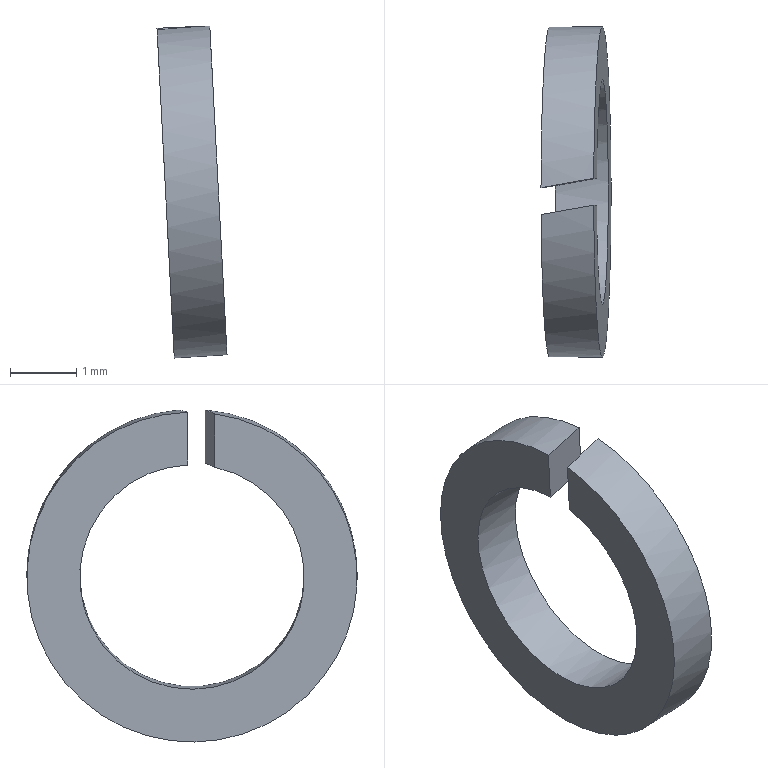Component | NX | GB93-87_3 | 1 solid | 6 faces | box 1.06 x 5 x 5.03 mm | volume 8 mm3 | plane 4 | cylinder 2 | commonest cylinder face diameters 5 x1 3.4 x1
STEP:
#1=CARTESIAN_POINT('',(0.,0.,0.));
#2=DIRECTION('',(0.,0.,1.));
#3=DIRECTION('',(1.,0.,0.));
#4=AXIS2_PLACEMENT_3D('',#1,#2,#3);
#5=CARTESIAN_POINT('',(4.816,-45.247,162.495));
#6=VERTEX_POINT('',#5);
#7=CARTESIAN_POINT('',(4.816,-44.841,162.495));
#8=VERTEX_POINT('',#7);
#9=CARTESIAN_POINT('',(4.947,-45.044,160.007));
#10=DIRECTION('',(0.9986,0.,0.05234));
#11=DIRECTION('',(0.05234,0.,-0.9986));
#12=AXIS2_PLACEMENT_3D('',#9,#10,#11);
#13=CIRCLE('',#12,2.5);
#14=CARTESIAN_POINT('',(4.947,-45.044,160.007));
#15=DIRECTION('',(0.9986,0.,0.05234));
#16=DIRECTION('',(0.05234,0.,-0.9986));
#17=AXIS2_PLACEMENT_3D('',#14,#15,#16);
#18=CYLINDRICAL_SURFACE('',#17,2.5);
#19=CARTESIAN_POINT('',(-6.283,0.));
#20=DIRECTION('',(1.,0.));
#21=VECTOR('',#20,1.);
#22=LINE('',#19,#21);
#23=(GEOMETRIC_REPRESENTATION_CONTEXT(2)PARAMETRIC_REPRESENTATION_CONTEXT()REPRESENTATION_CONTEXT('',''));
#24=DEFINITIONAL_REPRESENTATION('',(#22),#23);
#25=PCURVE('',#18,#24);
#26=CARTESIAN_POINT('',(4.947,-43.344,160.007));
#27=DIRECTION('',(0.9986,0.,0.05234));
#28=DIRECTION('',(0.05234,0.,-0.9986));
#29=AXIS2_PLACEMENT_3D('',#26,#27,#28);
#30=PLANE('',#29);
#31=CARTESIAN_POINT('',(0.,-1.7));
#32=DIRECTION('',(1.,0.));
#33=AXIS2_PLACEMENT_2D('',#31,#32);
#34=CIRCLE('',#33,2.5);
#35=(GEOMETRIC_REPRESENTATION_CONTEXT(2)PARAMETRIC_REPRESENTATION_CONTEXT()REPRESENTATION_CONTEXT('',''));
#36=DEFINITIONAL_REPRESENTATION('',(#34),#35);
#37=PCURVE('',#30,#36);
#38=SURFACE_CURVE('',#13,(#25,#37),.PCURVE_S1.);
#39=EDGE_CURVE('',#6,#8,#38,.T.);
#40=ORIENTED_EDGE('',*,*,#39,.F.);
#41=CARTESIAN_POINT('',(4.018,-45.388,162.438));
#42=VERTEX_POINT('',#41);
#43=CARTESIAN_POINT('',(6.097,-45.044,160.067));
#44=DIRECTION('',(0.1734,-0.9848,0.009088));
#45=DIRECTION('',(0.9835,0.1736,0.05154));
#46=AXIS2_PLACEMENT_3D('',#43,#44,#45);
#47=ELLIPSE('',#46,14.397,2.5);
#48=CARTESIAN_POINT('',(-3.06,-0.));
#49=CARTESIAN_POINT('',(-3.003,-0.8));
#50=B_SPLINE_CURVE_WITH_KNOTS('',1,(#48,#49),.UNSPECIFIED.,.F.,.F.,(2,2),(1.652,1.709),.PIECEWISE_BEZIER_KNOTS.);
#51=(GEOMETRIC_REPRESENTATION_CONTEXT(2)PARAMETRIC_REPRESENTATION_CONTEXT()REPRESENTATION_CONTEXT('',''));
#52=DEFINITIONAL_REPRESENTATION('',(#50),#51);
#53=PCURVE('',#18,#52);
#54=CARTESIAN_POINT('',(3.605,-45.449,163.692));
#55=DIRECTION('',(-0.1734,0.9848,-0.009088));
#56=DIRECTION('',(-0.9835,-0.1736,-0.05154));
#57=AXIS2_PLACEMENT_3D('',#54,#55,#56);
#58=PLANE('',#57);
#59=CARTESIAN_POINT('',(-16.731,-3.75));
#60=CARTESIAN_POINT('',(-16.731,0.5801));
#61=CARTESIAN_POINT('',(4.864,-1.585));
#62=CARTESIAN_POINT('',(26.46,-3.75));
#63=CARTESIAN_POINT('',(4.864,-5.915));
#64=CARTESIAN_POINT('',(-16.731,-8.08));
#65=CARTESIAN_POINT('',(-16.731,-3.75));
#66=(BOUNDED_CURVE()B_SPLINE_CURVE(2,(#59,#60,#61,#62,#63,#64,#65),.UNSPECIFIED.,.T.,.F.)B_SPLINE_CURVE_WITH_KNOTS((1,2,2,2,2,1),(-2.094,0.,2.094,4.189,6.283,8.378),.UNSPECIFIED.)CURVE()GEOMETRIC_REPRESENTATION_ITEM()RATIONAL_B_SPLINE_CURVE((1.,0.5,1.,0.5,1.,0.5,1.))REPRESENTATION_ITEM(''));
#67=(GEOMETRIC_REPRESENTATION_CONTEXT(2)PARAMETRIC_REPRESENTATION_CONTEXT()REPRESENTATION_CONTEXT('',''));
#68=DEFINITIONAL_REPRESENTATION('',(#66),#67);
#69=PCURVE('',#58,#68);
#70=SURFACE_CURVE('',#47,(#53,#69),.PCURVE_S1.);
#71=EDGE_CURVE('',#6,#42,#70,.T.);
#72=ORIENTED_EDGE('',*,*,#71,.T.);
#73=CARTESIAN_POINT('',(4.017,-44.982,162.461));
#74=VERTEX_POINT('',#73);
#75=CARTESIAN_POINT('',(4.148,-45.044,159.965));
#76=DIRECTION('',(0.9986,0.,0.05234));
#77=DIRECTION('',(0.05234,0.,-0.9986));
#78=AXIS2_PLACEMENT_3D('',#75,#76,#77);
#79=CIRCLE('',#78,2.5);
#80=CARTESIAN_POINT('',(-6.283,-0.8));
#81=DIRECTION('',(1.,-0.));
#82=VECTOR('',#81,1.);
#83=LINE('',#80,#82);
#84=(GEOMETRIC_REPRESENTATION_CONTEXT(2)PARAMETRIC_REPRESENTATION_CONTEXT()REPRESENTATION_CONTEXT('',''));
#85=DEFINITIONAL_REPRESENTATION('',(#83),#84);
#86=PCURVE('',#18,#85);
#87=CARTESIAN_POINT('',(4.148,-42.544,159.965));
#88=DIRECTION('',(-0.9986,0.,-0.05234));
#89=DIRECTION('',(-0.05234,0.,0.9986));
#90=AXIS2_PLACEMENT_3D('',#87,#88,#89);
#91=PLANE('',#90);
#92=CARTESIAN_POINT('',(-2.5,-2.5));
#93=CARTESIAN_POINT('',(-2.5,1.83));
#94=CARTESIAN_POINT('',(1.25,-0.3349));
#95=CARTESIAN_POINT('',(5.,-2.5));
#96=CARTESIAN_POINT('',(1.25,-4.665));
#97=CARTESIAN_POINT('',(-2.5,-6.83));
#98=CARTESIAN_POINT('',(-2.5,-2.5));
#99=(BOUNDED_CURVE()B_SPLINE_CURVE(2,(#92,#93,#94,#95,#96,#97,#98),.UNSPECIFIED.,.T.,.F.)B_SPLINE_CURVE_WITH_KNOTS((1,2,2,2,2,1),(-2.094,0.,2.094,4.189,6.283,8.378),.UNSPECIFIED.)CURVE()GEOMETRIC_REPRESENTATION_ITEM()RATIONAL_B_SPLINE_CURVE((1.,0.5,1.,0.5,1.,0.5,1.))REPRESENTATION_ITEM(''));
#100=(GEOMETRIC_REPRESENTATION_CONTEXT(2)PARAMETRIC_REPRESENTATION_CONTEXT()REPRESENTATION_CONTEXT('',''));
#101=DEFINITIONAL_REPRESENTATION('',(#99),#100);
#102=PCURVE('',#91,#101);
#103=SURFACE_CURVE('',#79,(#86,#102),.PCURVE_S1.);
#104=EDGE_CURVE('',#42,#74,#103,.T.);
#105=ORIENTED_EDGE('',*,*,#104,.T.);
#106=CARTESIAN_POINT('',(3.797,-45.044,159.947));
#107=DIRECTION('',(-0.1734,0.9848,-0.009088));
#108=DIRECTION('',(0.9835,0.1736,0.05154));
#109=AXIS2_PLACEMENT_3D('',#106,#107,#108);
#110=ELLIPSE('',#109,14.397,2.5);
#111=CARTESIAN_POINT('',(3.117,-0.8));
#112=CARTESIAN_POINT('',(3.06,-0.));
#113=B_SPLINE_CURVE_WITH_KNOTS('',1,(#111,#112),.UNSPECIFIED.,.F.,.F.,(2,2),(4.737,4.794),.PIECEWISE_BEZIER_KNOTS.);
#114=(GEOMETRIC_REPRESENTATION_CONTEXT(2)PARAMETRIC_REPRESENTATION_CONTEXT()REPRESENTATION_CONTEXT('',''));
#115=DEFINITIONAL_REPRESENTATION('',(#113),#114);
#116=PCURVE('',#18,#115);
#117=CARTESIAN_POINT('',(5.896,-44.638,163.812));
#118=DIRECTION('',(0.1734,-0.9848,0.009088));
#119=DIRECTION('',(0.9835,0.1736,0.05154));
#120=AXIS2_PLACEMENT_3D('',#117,#118,#119);
#121=PLANE('',#120);
#122=CARTESIAN_POINT('',(12.063,-3.75));
#123=CARTESIAN_POINT('',(12.063,-8.08));
#124=CARTESIAN_POINT('',(-9.533,-5.915));
#125=CARTESIAN_POINT('',(-31.128,-3.75));
#126=CARTESIAN_POINT('',(-9.533,-1.585));
#127=CARTESIAN_POINT('',(12.063,0.5801));
#128=CARTESIAN_POINT('',(12.063,-3.75));
#129=(BOUNDED_CURVE()B_SPLINE_CURVE(2,(#122,#123,#124,#125,#126,#127,#128),.UNSPECIFIED.,.T.,.F.)B_SPLINE_CURVE_WITH_KNOTS((1,2,2,2,2,1),(-2.094,0.,2.094,4.189,6.283,8.378),.UNSPECIFIED.)CURVE()GEOMETRIC_REPRESENTATION_ITEM()RATIONAL_B_SPLINE_CURVE((1.,0.5,1.,0.5,1.,0.5,1.))REPRESENTATION_ITEM(''));
#130=(GEOMETRIC_REPRESENTATION_CONTEXT(2)PARAMETRIC_REPRESENTATION_CONTEXT()REPRESENTATION_CONTEXT('',''));
#131=DEFINITIONAL_REPRESENTATION('',(#129),#130);
#132=PCURVE('',#121,#131);
#133=SURFACE_CURVE('',#110,(#116,#132),.PCURVE_S1.);
#134=EDGE_CURVE('',#74,#8,#133,.T.);
#135=ORIENTED_EDGE('',*,*,#134,.T.);
#136=EDGE_LOOP('',(#40,#72,#105,#135));
#137=FACE_BOUND('',#136,.T.);
#138=ADVANCED_FACE('',(#137),#18,.T.);
#139=ORIENTED_EDGE('',*,*,#104,.F.);
#140=CARTESIAN_POINT('',(4.061,-45.388,161.628));
#141=VERTEX_POINT('',#140);
#142=CARTESIAN_POINT('',(4.148,-45.388,159.965));
#143=DIRECTION('',(0.05234,0.,-0.9986));
#144=VECTOR('',#143,1.);
#145=LINE('',#142,#144);
#146=CARTESIAN_POINT('',(0.,-2.844));
#147=DIRECTION('',(-1.,0.));
#148=VECTOR('',#147,1.);
#149=LINE('',#146,#148);
#150=(GEOMETRIC_REPRESENTATION_CONTEXT(2)PARAMETRIC_REPRESENTATION_CONTEXT()REPRESENTATION_CONTEXT('',''));
#151=DEFINITIONAL_REPRESENTATION('',(#149),#150);
#152=PCURVE('',#91,#151);
#153=CARTESIAN_POINT('',(-0.3524,-3.75));
#154=DIRECTION('',(-0.,-1.));
#155=VECTOR('',#154,1.);
#156=LINE('',#153,#155);
#157=(GEOMETRIC_REPRESENTATION_CONTEXT(2)PARAMETRIC_REPRESENTATION_CONTEXT()REPRESENTATION_CONTEXT('',''));
#158=DEFINITIONAL_REPRESENTATION('',(#156),#157);
#159=PCURVE('',#58,#158);
#160=SURFACE_CURVE('',#145,(#152,#159),.PCURVE_S1.);
#161=EDGE_CURVE('',#42,#141,#160,.T.);
#162=ORIENTED_EDGE('',*,*,#161,.T.);
#163=CARTESIAN_POINT('',(4.059,-44.982,161.662));
#164=VERTEX_POINT('',#163);
#165=CARTESIAN_POINT('',(4.148,-45.044,159.965));
#166=DIRECTION('',(0.9986,0.,0.05234));
#167=DIRECTION('',(0.05234,0.,-0.9986));
#168=AXIS2_PLACEMENT_3D('',#165,#166,#167);
#169=CIRCLE('',#168,1.7);
#170=CARTESIAN_POINT('',(-1.7,-2.5));
#171=CARTESIAN_POINT('',(-1.7,0.4445));
#172=CARTESIAN_POINT('',(0.85,-1.028));
#173=CARTESIAN_POINT('',(3.4,-2.5));
#174=CARTESIAN_POINT('',(0.85,-3.972));
#175=CARTESIAN_POINT('',(-1.7,-5.444));
#176=CARTESIAN_POINT('',(-1.7,-2.5));
#177=(BOUNDED_CURVE()B_SPLINE_CURVE(2,(#170,#171,#172,#173,#174,#175,#176),.UNSPECIFIED.,.T.,.F.)B_SPLINE_CURVE_WITH_KNOTS((1,2,2,2,2,1),(-2.094,0.,2.094,4.189,6.283,8.378),.UNSPECIFIED.)CURVE()GEOMETRIC_REPRESENTATION_ITEM()RATIONAL_B_SPLINE_CURVE((1.,0.5,1.,0.5,1.,0.5,1.))REPRESENTATION_ITEM(''));
#178=(GEOMETRIC_REPRESENTATION_CONTEXT(2)PARAMETRIC_REPRESENTATION_CONTEXT()REPRESENTATION_CONTEXT('',''));
#179=DEFINITIONAL_REPRESENTATION('',(#177),#178);
#180=PCURVE('',#91,#179);
#181=CARTESIAN_POINT('',(4.947,-45.044,160.007));
#182=DIRECTION('',(0.9986,0.,0.05234));
#183=DIRECTION('',(0.05234,0.,-0.9986));
#184=AXIS2_PLACEMENT_3D('',#181,#182,#183);
#185=CYLINDRICAL_SURFACE('',#184,1.7);
#186=CARTESIAN_POINT('',(-6.283,-0.8));
#187=DIRECTION('',(1.,-0.));
#188=VECTOR('',#187,1.);
#189=LINE('',#186,#188);
#190=(GEOMETRIC_REPRESENTATION_CONTEXT(2)PARAMETRIC_REPRESENTATION_CONTEXT()REPRESENTATION_CONTEXT('',''));
#191=DEFINITIONAL_REPRESENTATION('',(#189),#190);
#192=PCURVE('',#185,#191);
#193=SURFACE_CURVE('',#169,(#180,#192),.PCURVE_S1.);
#194=EDGE_CURVE('',#141,#164,#193,.T.);
#195=ORIENTED_EDGE('',*,*,#194,.T.);
#196=CARTESIAN_POINT('',(4.148,-44.982,159.965));
#197=DIRECTION('',(-0.05234,0.,0.9986));
#198=VECTOR('',#197,1.);
#199=LINE('',#196,#198);
#200=CARTESIAN_POINT('',(0.,-2.438));
#201=DIRECTION('',(1.,0.));
#202=VECTOR('',#201,1.);
#203=LINE('',#200,#202);
#204=(GEOMETRIC_REPRESENTATION_CONTEXT(2)PARAMETRIC_REPRESENTATION_CONTEXT()REPRESENTATION_CONTEXT('',''));
#205=DEFINITIONAL_REPRESENTATION('',(#203),#204);
#206=PCURVE('',#91,#205);
#207=CARTESIAN_POINT('',(-1.977,-3.75));
#208=DIRECTION('',(-0.,1.));
#209=VECTOR('',#208,1.);
#210=LINE('',#207,#209);
#211=(GEOMETRIC_REPRESENTATION_CONTEXT(2)PARAMETRIC_REPRESENTATION_CONTEXT()REPRESENTATION_CONTEXT('',''));
#212=DEFINITIONAL_REPRESENTATION('',(#210),#211);
#213=PCURVE('',#121,#212);
#214=SURFACE_CURVE('',#199,(#206,#213),.PCURVE_S1.);
#215=EDGE_CURVE('',#164,#74,#214,.T.);
#216=ORIENTED_EDGE('',*,*,#215,.T.);
#217=EDGE_LOOP('',(#139,#162,#195,#216));
#218=FACE_BOUND('',#217,.T.);
#219=ADVANCED_FACE('',(#218),#91,.T.);
#220=CARTESIAN_POINT('',(4.859,-44.841,161.693));
#221=VERTEX_POINT('',#220);
#222=CARTESIAN_POINT('',(3.797,-45.044,159.947));
#223=DIRECTION('',(0.1734,-0.9848,0.009088));
#224=DIRECTION('',(0.9835,0.1736,0.05154));
#225=AXIS2_PLACEMENT_3D('',#222,#223,#224);
#226=ELLIPSE('',#225,9.79,1.7);
#227=CARTESIAN_POINT('',(3.022,-0.));
#228=CARTESIAN_POINT('',(3.105,-0.8));
#229=B_SPLINE_CURVE_WITH_KNOTS('',1,(#227,#228),.UNSPECIFIED.,.F.,.F.,(2,2),(1.451,1.534),.PIECEWISE_BEZIER_KNOTS.);
#230=(GEOMETRIC_REPRESENTATION_CONTEXT(2)PARAMETRIC_REPRESENTATION_CONTEXT()REPRESENTATION_CONTEXT('',''));
#231=DEFINITIONAL_REPRESENTATION('',(#229),#230);
#232=PCURVE('',#185,#231);
#233=CARTESIAN_POINT('',(-2.334,-3.75));
#234=DIRECTION('',(1.,0.));
#235=AXIS2_PLACEMENT_2D('',#233,#234);
#236=ELLIPSE('',#235,9.79,1.7);
#237=(GEOMETRIC_REPRESENTATION_CONTEXT(2)PARAMETRIC_REPRESENTATION_CONTEXT()REPRESENTATION_CONTEXT('',''));
#238=DEFINITIONAL_REPRESENTATION('',(#236),#237);
#239=PCURVE('',#121,#238);
#240=SURFACE_CURVE('',#226,(#232,#239),.PCURVE_S1.);
#241=EDGE_CURVE('',#221,#164,#240,.T.);
#242=ORIENTED_EDGE('',*,*,#241,.F.);
#243=CARTESIAN_POINT('',(4.859,-45.247,161.693));
#244=VERTEX_POINT('',#243);
#245=CARTESIAN_POINT('',(4.947,-45.044,160.007));
#246=DIRECTION('',(0.9986,0.,0.05234));
#247=DIRECTION('',(0.05234,0.,-0.9986));
#248=AXIS2_PLACEMENT_3D('',#245,#246,#247);
#249=CIRCLE('',#248,1.7);
#250=CARTESIAN_POINT('',(-6.283,-0.));
#251=DIRECTION('',(1.,0.));
#252=VECTOR('',#251,1.);
#253=LINE('',#250,#252);
#254=(GEOMETRIC_REPRESENTATION_CONTEXT(2)PARAMETRIC_REPRESENTATION_CONTEXT()REPRESENTATION_CONTEXT('',''));
#255=DEFINITIONAL_REPRESENTATION('',(#253),#254);
#256=PCURVE('',#185,#255);
#257=CARTESIAN_POINT('',(0.,-1.7));
#258=DIRECTION('',(1.,0.));
#259=AXIS2_PLACEMENT_2D('',#257,#258);
#260=CIRCLE('',#259,1.7);
#261=(GEOMETRIC_REPRESENTATION_CONTEXT(2)PARAMETRIC_REPRESENTATION_CONTEXT()REPRESENTATION_CONTEXT('',''));
#262=DEFINITIONAL_REPRESENTATION('',(#260),#261);
#263=PCURVE('',#30,#262);
#264=SURFACE_CURVE('',#249,(#256,#263),.PCURVE_S1.);
#265=EDGE_CURVE('',#244,#221,#264,.T.);
#266=ORIENTED_EDGE('',*,*,#265,.F.);
#267=CARTESIAN_POINT('',(6.097,-45.044,160.067));
#268=DIRECTION('',(-0.1734,0.9848,-0.009088));
#269=DIRECTION('',(0.9835,0.1736,0.05154));
#270=AXIS2_PLACEMENT_3D('',#267,#268,#269);
#271=ELLIPSE('',#270,9.79,1.7);
#272=CARTESIAN_POINT('',(-2.938,-0.8));
#273=CARTESIAN_POINT('',(-3.022,-0.));
#274=B_SPLINE_CURVE_WITH_KNOTS('',1,(#272,#273),.UNSPECIFIED.,.F.,.F.,(2,2),(4.509,4.593),.PIECEWISE_BEZIER_KNOTS.);
#275=(GEOMETRIC_REPRESENTATION_CONTEXT(2)PARAMETRIC_REPRESENTATION_CONTEXT()REPRESENTATION_CONTEXT('',''));
#276=DEFINITIONAL_REPRESENTATION('',(#274),#275);
#277=PCURVE('',#185,#276);
#278=CARTESIAN_POINT('',(-2.334,-3.75));
#279=DIRECTION('',(-1.,0.));
#280=AXIS2_PLACEMENT_2D('',#278,#279);
#281=ELLIPSE('',#280,9.79,1.7);
#282=(GEOMETRIC_REPRESENTATION_CONTEXT(2)PARAMETRIC_REPRESENTATION_CONTEXT()REPRESENTATION_CONTEXT('',''));
#283=DEFINITIONAL_REPRESENTATION('',(#281),#282);
#284=PCURVE('',#58,#283);
#285=SURFACE_CURVE('',#271,(#277,#284),.PCURVE_S1.);
#286=EDGE_CURVE('',#141,#244,#285,.T.);
#287=ORIENTED_EDGE('',*,*,#286,.F.);
#288=ORIENTED_EDGE('',*,*,#194,.T.);
#289=EDGE_LOOP('',(#242,#266,#287,#288));
#290=FACE_BOUND('',#289,.F.);
#291=ADVANCED_FACE('',(#290),#185,.F.);
#292=ORIENTED_EDGE('',*,*,#265,.F.);
#293=CARTESIAN_POINT('',(4.947,-45.247,160.007));
#294=DIRECTION('',(-0.05234,0.,0.9986));
#295=VECTOR('',#294,1.);
#296=LINE('',#293,#295);
#297=CARTESIAN_POINT('',(0.,-1.903));
#298=DIRECTION('',(-1.,0.));
#299=VECTOR('',#298,1.);
#300=LINE('',#297,#299);
#301=(GEOMETRIC_REPRESENTATION_CONTEXT(2)PARAMETRIC_REPRESENTATION_CONTEXT()REPRESENTATION_CONTEXT('',''));
#302=DEFINITIONAL_REPRESENTATION('',(#300),#301);
#303=PCURVE('',#30,#302);
#304=CARTESIAN_POINT('',(-1.165,-3.75));
#305=DIRECTION('',(0.,1.));
#306=VECTOR('',#305,1.);
#307=LINE('',#304,#306);
#308=(GEOMETRIC_REPRESENTATION_CONTEXT(2)PARAMETRIC_REPRESENTATION_CONTEXT()REPRESENTATION_CONTEXT('',''));
#309=DEFINITIONAL_REPRESENTATION('',(#307),#308);
#310=PCURVE('',#58,#309);
#311=SURFACE_CURVE('',#296,(#303,#310),.PCURVE_S1.);
#312=EDGE_CURVE('',#244,#6,#311,.T.);
#313=ORIENTED_EDGE('',*,*,#312,.T.);
#314=ORIENTED_EDGE('',*,*,#39,.T.);
#315=CARTESIAN_POINT('',(4.947,-44.841,160.007));
#316=DIRECTION('',(0.05234,0.,-0.9986));
#317=VECTOR('',#316,1.);
#318=LINE('',#315,#317);
#319=CARTESIAN_POINT('',(0.,-1.497));
#320=DIRECTION('',(1.,0.));
#321=VECTOR('',#320,1.);
#322=LINE('',#319,#321);
#323=(GEOMETRIC_REPRESENTATION_CONTEXT(2)PARAMETRIC_REPRESENTATION_CONTEXT()REPRESENTATION_CONTEXT('',''));
#324=DEFINITIONAL_REPRESENTATION('',(#322),#323);
#325=PCURVE('',#30,#324);
#326=CARTESIAN_POINT('',(-1.165,-3.75));
#327=DIRECTION('',(0.,-1.));
#328=VECTOR('',#327,1.);
#329=LINE('',#326,#328);
#330=(GEOMETRIC_REPRESENTATION_CONTEXT(2)PARAMETRIC_REPRESENTATION_CONTEXT()REPRESENTATION_CONTEXT('',''));
#331=DEFINITIONAL_REPRESENTATION('',(#329),#330);
#332=PCURVE('',#121,#331);
#333=SURFACE_CURVE('',#318,(#325,#332),.PCURVE_S1.);
#334=EDGE_CURVE('',#8,#221,#333,.T.);
#335=ORIENTED_EDGE('',*,*,#334,.T.);
#336=EDGE_LOOP('',(#292,#313,#314,#335));
#337=FACE_BOUND('',#336,.T.);
#338=ADVANCED_FACE('',(#337),#30,.T.);
#339=ORIENTED_EDGE('',*,*,#215,.F.);
#340=ORIENTED_EDGE('',*,*,#241,.F.);
#341=ORIENTED_EDGE('',*,*,#334,.F.);
#342=ORIENTED_EDGE('',*,*,#134,.F.);
#343=EDGE_LOOP('',(#339,#340,#341,#342));
#344=FACE_BOUND('',#343,.T.);
#345=ADVANCED_FACE('',(#344),#121,.T.);
#346=ORIENTED_EDGE('',*,*,#312,.F.);
#347=ORIENTED_EDGE('',*,*,#286,.F.);
#348=ORIENTED_EDGE('',*,*,#161,.F.);
#349=ORIENTED_EDGE('',*,*,#71,.F.);
#350=EDGE_LOOP('',(#346,#347,#348,#349));
#351=FACE_BOUND('',#350,.T.);
#352=ADVANCED_FACE('',(#351),#58,.T.);
#353=CLOSED_SHELL('',(#138,#219,#291,#338,#345,#352));
#354=MANIFOLD_SOLID_BREP('',#353);
#355=(LENGTH_UNIT()NAMED_UNIT(*)SI_UNIT(.MILLI.,.METRE.));
#356=UNCERTAINTY_MEASURE_WITH_UNIT(LENGTH_MEASURE(0.0005),#355,'','');
#357=(NAMED_UNIT(*)PLANE_ANGLE_UNIT()SI_UNIT($,.RADIAN.));
#358=(NAMED_UNIT(*)SI_UNIT($,.STERADIAN.)SOLID_ANGLE_UNIT());
#359=(GEOMETRIC_REPRESENTATION_CONTEXT(3)GLOBAL_UNCERTAINTY_ASSIGNED_CONTEXT((#356))GLOBAL_UNIT_ASSIGNED_CONTEXT((#355,#357,#358))REPRESENTATION_CONTEXT('',''));
#360=ADVANCED_BREP_SHAPE_REPRESENTATION('',(#4,#354),#359);